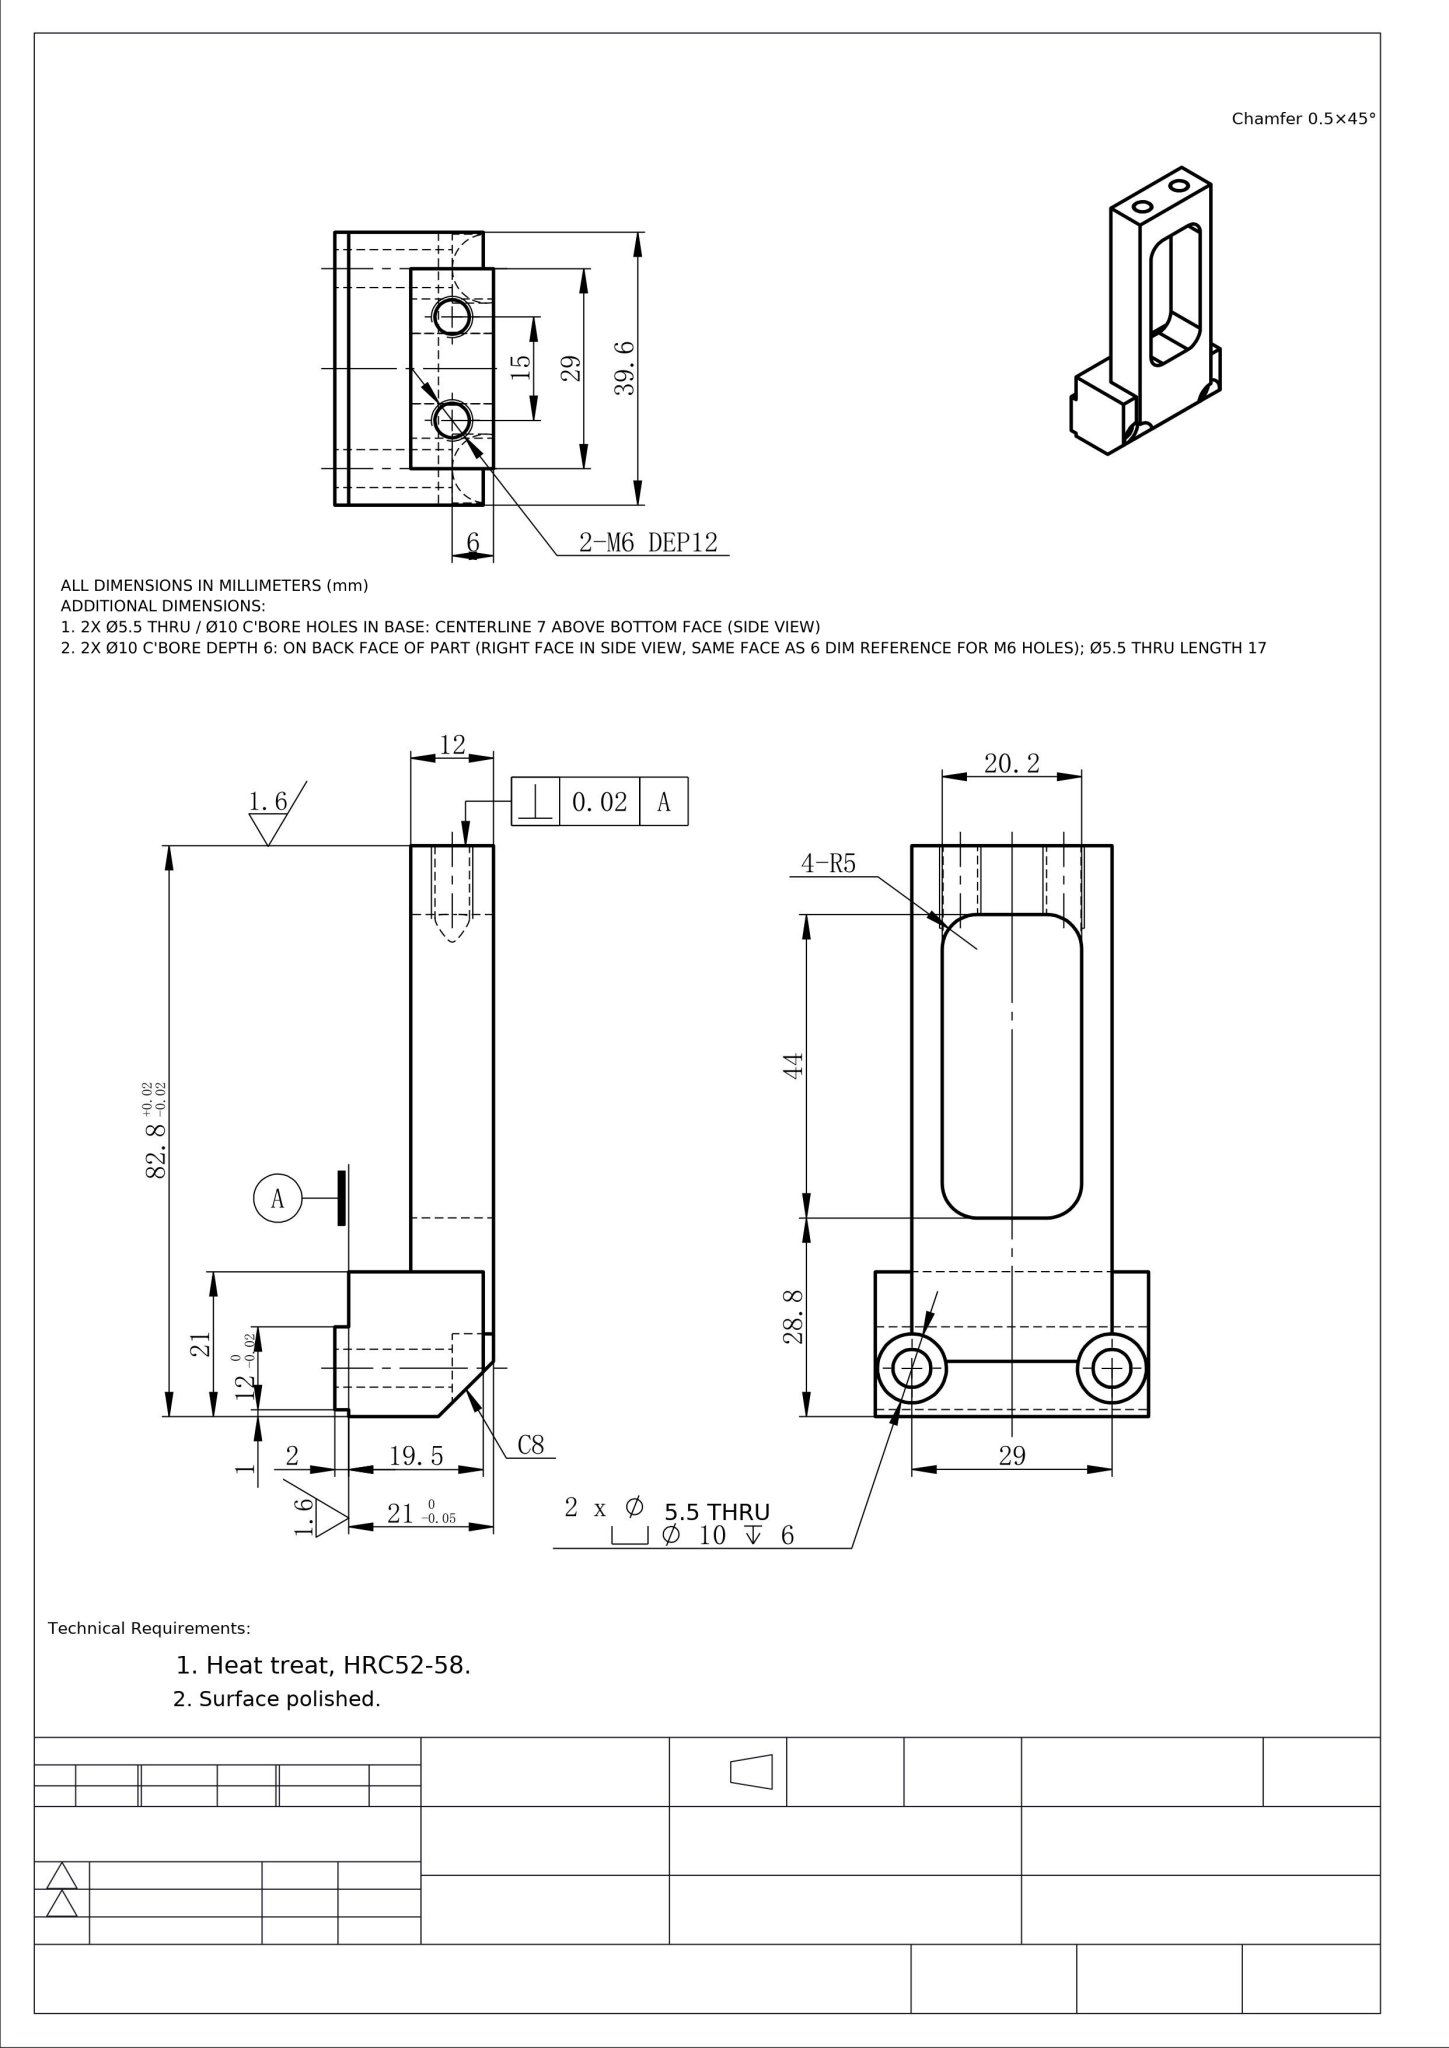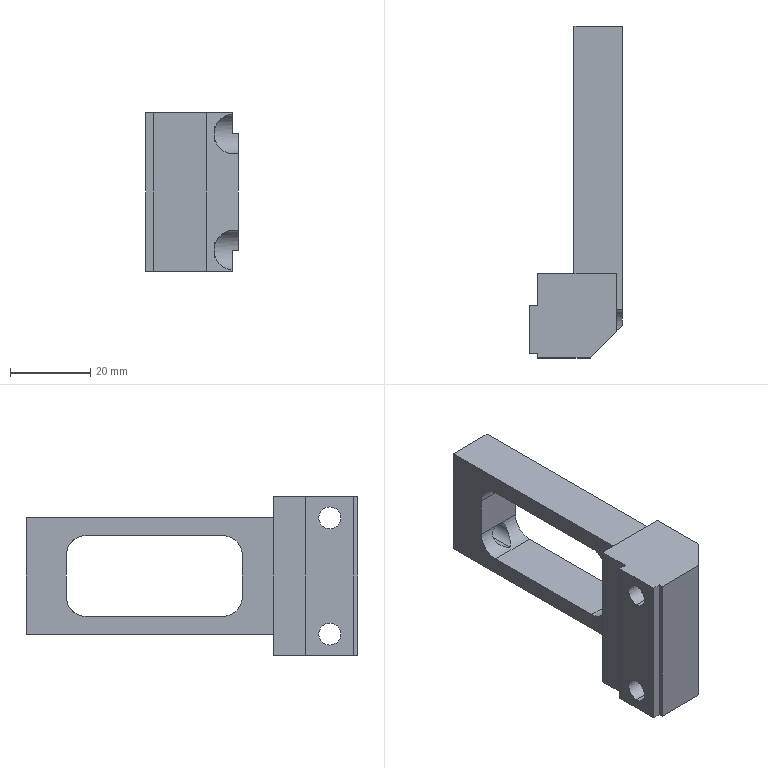Part | NX | mm | 1 solid | 41 faces | box 23 x 82.8 x 39.6 mm | volume 26159 mm3 | plane 23 | cylinder 18 | commonest cylinder face diameters 10 x10 5.5 x4 5 x4